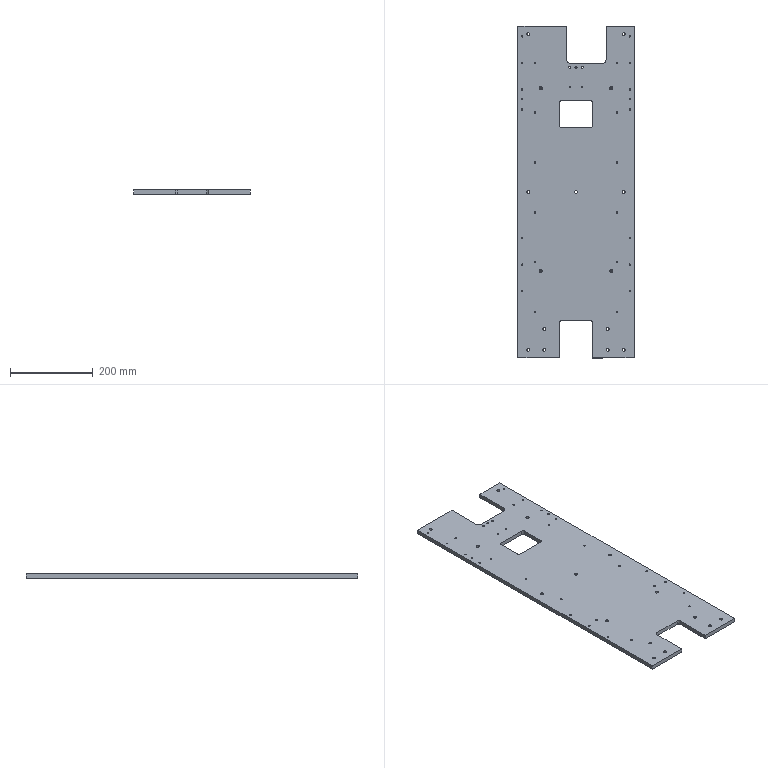Component | SolidWorks | DC-024-40-1 | 1 solid | 138 faces | box 280 x 800 x 10 mm | volume 2020777 mm3 | cylinder 112 | plane 18 | cone 8 | commonest cylinder face diameters 4.2 x32 3.3 x28 6.8 x22 4.5 x8 8 x8 5 x6 10 x6 20 x2
build123d program:
from build123d import *

# Parameters (mm, degrees)
SKETCH1_W                     = 280
SKETCH1_H                     = 860
BOSS_EXTRUDE1_DEPTH           = 5
SKETCH2_W                     = 80
SKETCH2_H                     = 180
CUT_EXTRUDE1_DEPTH            = 36
SKETCH3_W                     = 45
SKETCH3_H                     = 91
CUT_EXTRUDE2_DEPTH            = 36
SKETCH5_W                     = 50
SKETCH5_H                     = 91
CUT_EXTRUDE4_DEPTH            = 60
M4_TAPPED_HOLE1_D             = 3.3
FILLET1_R                     = 10
M5_TAPPED_HOLE1_D             = 4.2
M8_TAPPED_HOLE1_D             = 6.8
FILLET2_R                     = 5
M6_TAPPED_HOLE1_D             = 5
SIZE_MM_DOWEL_PIN_HOLE1_D     = 8
SIZE_MM_DOWEL_PIN_HOLE1_DEPTH = 6
SIZE_MM_DOWEL_PIN_HOLE1_TIP   = 2.403
F_4_5_4_5_DIAMETER_HOLE1_D    = 4.5
M5_TAPPED_HOLE2_D             = 4.2
M4_TAPPED_HOLE2_D             = 3.3
SKETCH26_W                    = 80
SKETCH26_H                    = 65
CUT_EXTRUDE5_DEPTH            = 20
FILLET3_R                     = 5
CUT_EXTRUDE6_DEPTH            = 127
CUT_EXTRUDE6_DEPTH_BACK       = 76
SKETCH28_W                    = 280
SKETCH28_H                    = 60
M8_TAPPED_HOLE2_D             = 6.8


with BuildPart() as part:
    # Sketch1 → Boss-Extrude1 (new, symmetric)
    with BuildSketch(Plane.XY):
        Rectangle(SKETCH1_W, SKETCH1_H)
    extrude(amount=BOSS_EXTRUDE1_DEPTH, both=True)

    # Sketch2 → Cut-Extrude1 (cut)
    with BuildSketch(Plane(origin=(0, 0, -5), x_dir=(-1, 0, 0), z_dir=(0, 0, -1))):
        with Locations((0, -430)):
            Rectangle(SKETCH2_W, SKETCH2_H)
    extrude(amount=-CUT_EXTRUDE1_DEPTH, mode=Mode.SUBTRACT)

    # Sketch3 → Cut-Extrude2 (cut)
    with BuildSketch(Plane.XY.offset(5)):
        with Locations((0, 324.5)):
            Rectangle(SKETCH3_W, SKETCH3_H)
    extrude(amount=-CUT_EXTRUDE2_DEPTH, mode=Mode.SUBTRACT)

    # Sketch5 → Cut-Extrude4 (cut)
    with BuildSketch(Plane.XY.offset(5)):
        with Locations((47.5, 324.5)):
            Rectangle(SKETCH5_W, SKETCH5_H)
    extrude(amount=-CUT_EXTRUDE4_DEPTH, mode=Mode.SUBTRACT)

    # M4 Tapped Hole1 (through all)
    with Locations(Plane.XY.offset(5)):
        with Locations((-14, 222.5), (14, 222.5)):
            Hole(M4_TAPPED_HOLE1_D / 2)

    # Fillet1
    fillet1_edges = [part.edges().sort_by_distance(p)[0] for p in [
        (-22.5, 279, 0),
        (72.5, 279, 0),
    ]]
    fillet(fillet1_edges, radius=FILLET1_R)

    # M5 Tapped Hole1 (through all)
    with Locations(Plane.XY.offset(5)):
        with Locations((-99, 281), (-99, 161), (-99, 41), (-99, -79), (-99, -199), (-99, -319), (99, -319), (99, -199), (99, -79), (99, 41), (99, 161), (99, 281)):
            Hole(M5_TAPPED_HOLE1_D / 2)

    # M8 Tapped Hole1 (through all)
    with Locations(Plane.XY.offset(5)):
        with Locations((76.5, -360), (-76.5, -360), (-76.5, -410), (76.5, -410)):
            Hole(M8_TAPPED_HOLE1_D / 2)

    # Fillet2
    fillet2_edges = [part.edges().sort_by_distance(p)[0] for p in [
        (-40, -340, 0),
        (40, -340, 0),
    ]]
    fillet(fillet2_edges, radius=FILLET2_R)

    # M6 Tapped Hole1 (through all)
    with Locations(Plane.XY.offset(5)):
        with Locations((15, 270.5), (-15, 270.5), (0, 270.5)):
            Hole(M6_TAPPED_HOLE1_D / 2)

    # Size mm Dowel Pin Hole1
    with Locations(Plane.XY.offset(5)):
        with Locations((-85, 220), (-85, -220), (85, 220), (85, -220)):
            Hole(SIZE_MM_DOWEL_PIN_HOLE1_D / 2, depth=SIZE_MM_DOWEL_PIN_HOLE1_DEPTH)
            with Locations((0, 0, -(SIZE_MM_DOWEL_PIN_HOLE1_DEPTH + SIZE_MM_DOWEL_PIN_HOLE1_TIP / 2))):  # 118° drill point
                Cone(0, SIZE_MM_DOWEL_PIN_HOLE1_D / 2, SIZE_MM_DOWEL_PIN_HOLE1_TIP, mode=Mode.SUBTRACT)

    # 4.5 _4.5_ Diameter Hole1 (through all)
    with Locations(Plane.XY.offset(5)):
        with Locations((-85, 220), (85, 220), (-85, -220), (85, -220)):
            Hole(F_4_5_4_5_DIAMETER_HOLE1_D / 2)

    # M5 Tapped Hole2 (through all)
    with Locations(Plane.XY.offset(5)):
        with Locations((130, 194), (130, 168)):
            m5_tapped_hole2 = Hole(M5_TAPPED_HOLE2_D / 2)

    # M4 Tapped Hole2 (through all)
    with Locations(Plane.XY.offset(5)):
        with Locations((129.5, 345), (129.5, 281), (129.5, 217), (129.5, -141), (129.5, -205), (129.5, -269)):
            m4_tapped_hole2 = Hole(M4_TAPPED_HOLE2_D / 2)

    # Sketch26 → Cut-Extrude5 (cut)
    with BuildSketch(Plane.XY.offset(5)):
        with Locations((0, 157.5)):
            Rectangle(SKETCH26_W, SKETCH26_H)
    extrude(amount=-CUT_EXTRUDE5_DEPTH, mode=Mode.SUBTRACT)

    # Fillet3
    fillet3_edges = [part.edges().sort_by_distance(p)[0] for p in [
        (40, 190, 0),
        (40, 125, 0),
        (-40, 125, 0),
        (-40, 190, 0),
    ]]
    fillet(fillet3_edges, radius=FILLET3_R)

    # Sketch28 → Cut-Extrude6 (cut, two sides: drawn at the far end of the back side and taken through both)
    with BuildSketch(Plane.XY.offset(5).offset(-CUT_EXTRUDE6_DEPTH_BACK)):
        with Locations((0, 400)):
            Rectangle(SKETCH28_W, SKETCH28_H)
    extrude(amount=CUT_EXTRUDE6_DEPTH + CUT_EXTRUDE6_DEPTH_BACK, mode=Mode.SUBTRACT)

    # M8 Tapped Hole2 (through all)
    with Locations(Plane.XY.offset(5)):
        with Locations((-115, -410), (115, -410), (115, -30), (0, -30), (-115, -30), (-115, 350), (115, 350)):
            Hole(M8_TAPPED_HOLE2_D / 2)

    # Mirror1: M5 Tapped Hole2, M4 Tapped Hole2 across plane
    add(m5_tapped_hole2.mirror(Plane(origin=(0, 0, 0), x_dir=(0, 0, 1), z_dir=(1, 0, 0))), mode=Mode.SUBTRACT)
    add(m4_tapped_hole2.mirror(Plane(origin=(0, 0, 0), x_dir=(0, 0, 1), z_dir=(1, 0, 0))), mode=Mode.SUBTRACT)


solid = part.part

# Placed as in the assembly
solid = solid.moved(Location((-25.633, -9.091, 8), (0, 0, 0)))